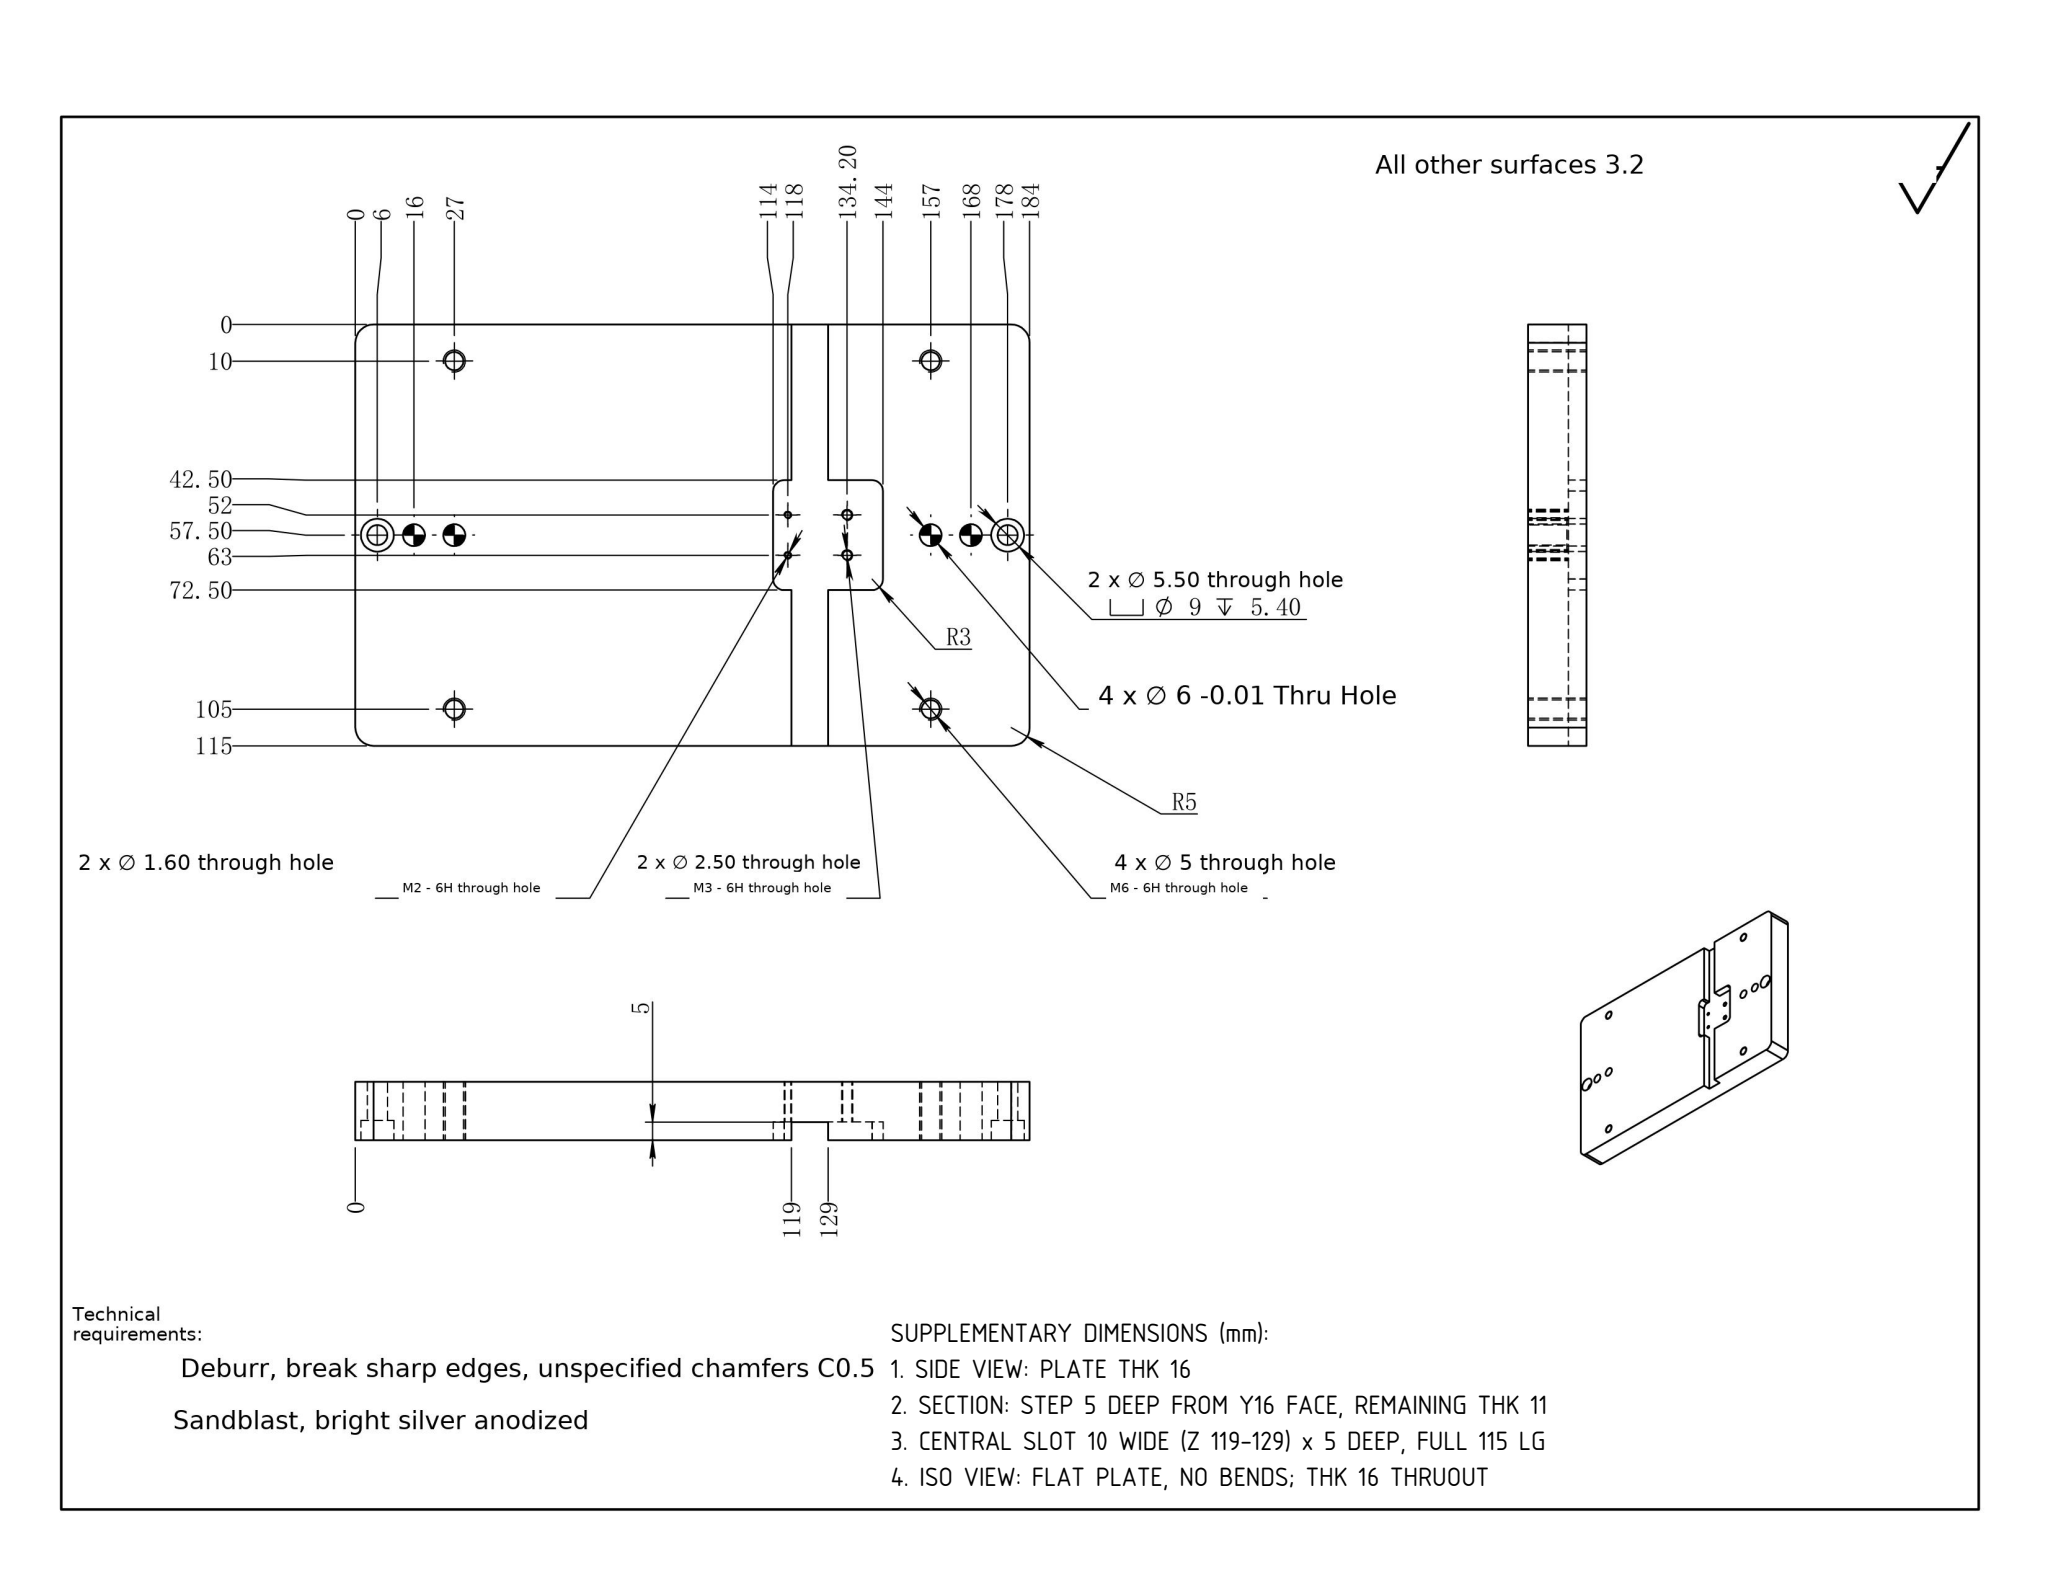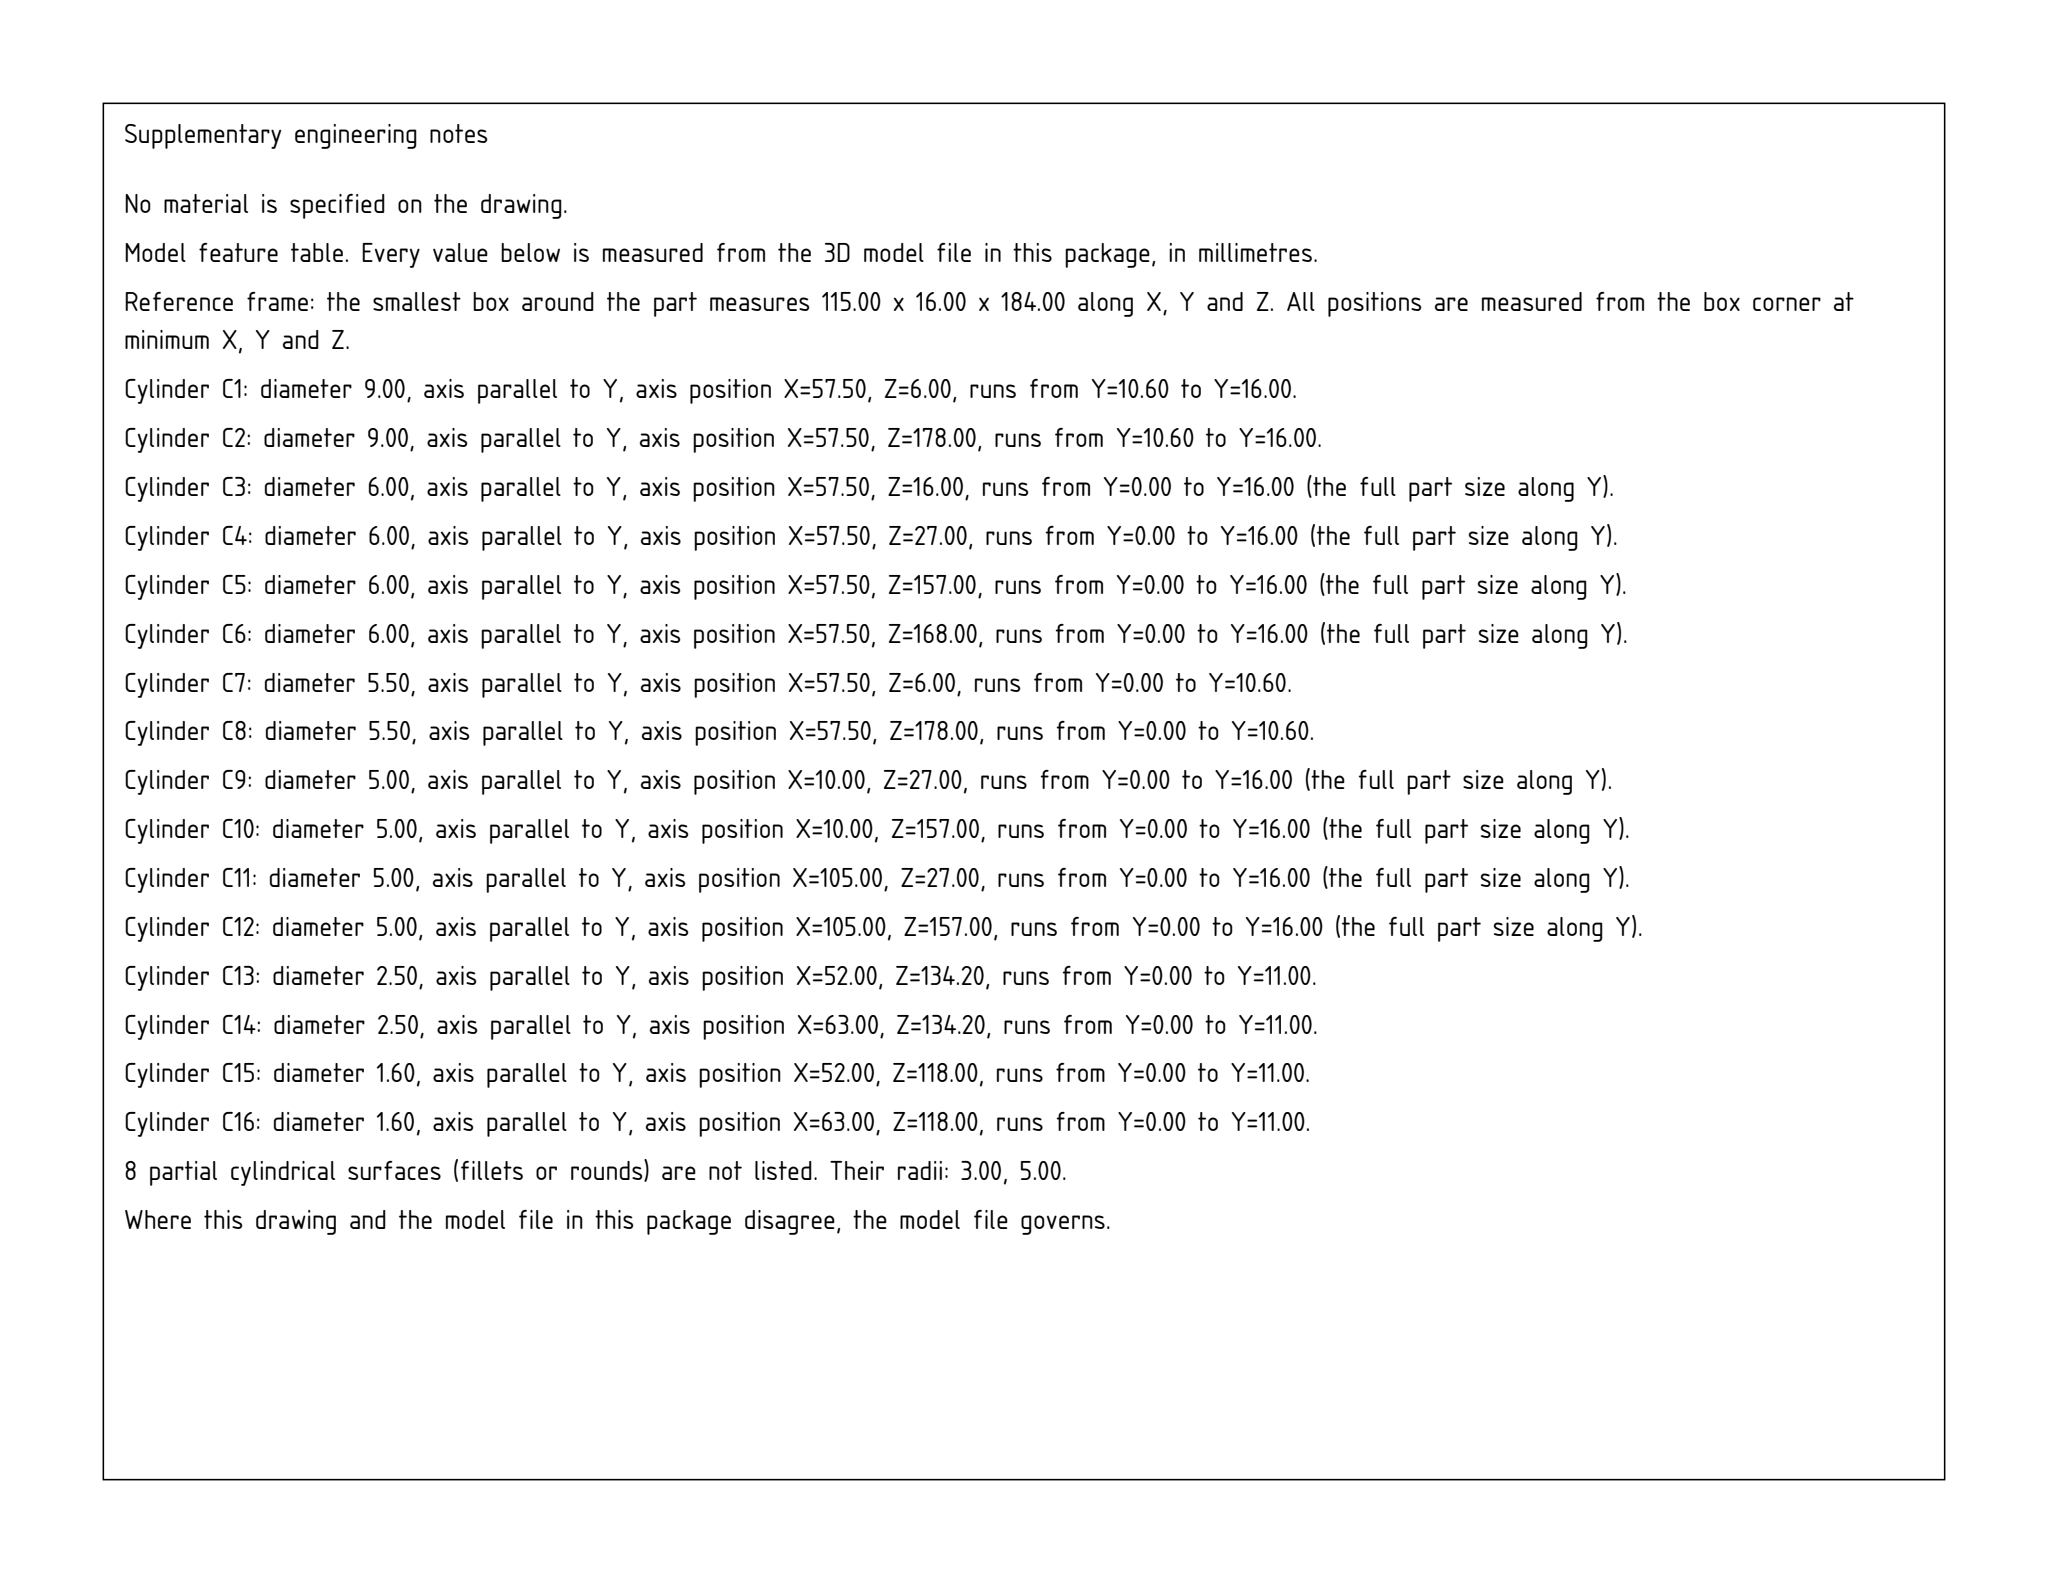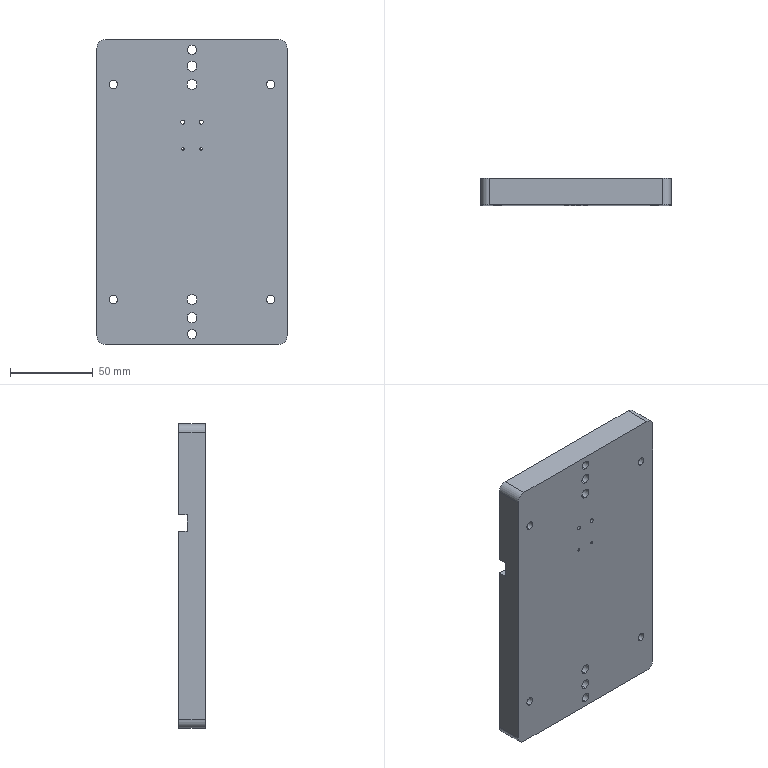Part | SolidWorks | mm | 1 solid | 60 faces | box 115 x 16 x 184 mm | volume 325096 mm3 | cylinder 40 | plane 20 | commonest cylinder face diameters 6 x12 5 x8 2.5 x4 1.6 x4 9 x4 5.5 x4 10 x4